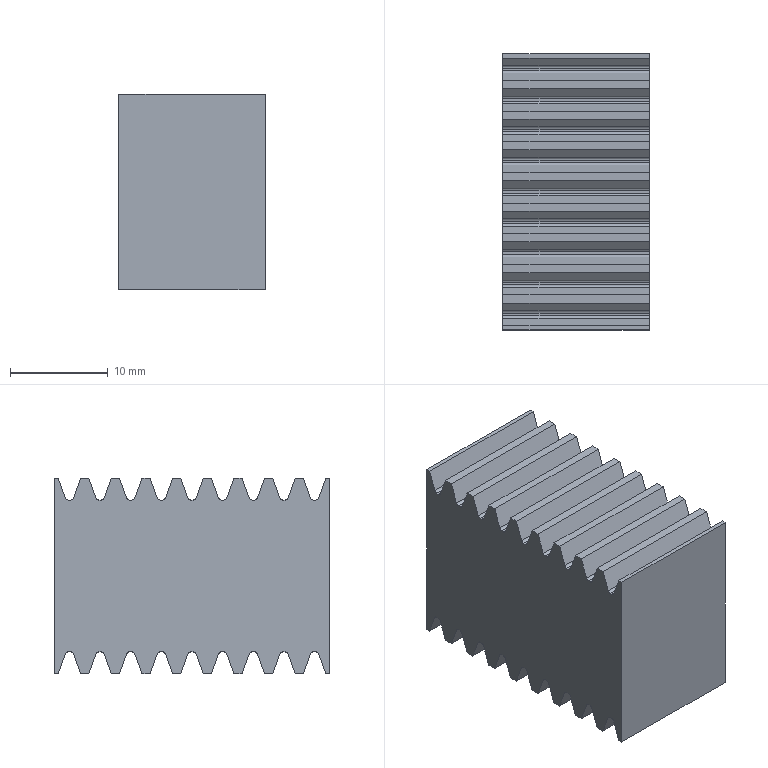Component | SolidWorks | ArmGrippingRack-1 | 1 solid | 117 faces | box 15.02 x 28.27 x 20.07 mm | volume 6038 mm3 | plane 79 | cylinder 38 | commonest cylinder face diameters 0.6 x36 10 x2
build123d program:
from build123d import *

# Parameters (mm, degrees)
EXTRUDECI_DEPTH                = 7.5
EXTRUDECI_DEPTH_BACK           = 7.5
SKETCHCI_M_STRSKETCHNAME_W     = 20.05
SKETCHCI_M_STRSKETCHNAME_H     = 69.115
TOOTHEXTRUDECUTSPURGEAR2_DEPTH = 7.5
PATTERNSPURGEAR2_COUNT         = 22
PATTERNSPURGEAR2_PITCH         = 3.142
MIRROR1_COPY_1_DEPTH           = 7.5
MIRROR1_COPY_2_DEPTH           = 7.5
MIRROR1_COPY_3_DEPTH           = 7.5
MIRROR1_COPY_4_DEPTH           = 7.5
MIRROR1_COPY_5_DEPTH           = 7.5
MIRROR1_COPY_6_DEPTH           = 7.5
MIRROR1_COPY_7_DEPTH           = 7.5
MIRROR1_COPY_8_DEPTH           = 7.5
MIRROR1_COPY_9_DEPTH           = 7.5
MIRROR1_COPY_10_DEPTH          = 7.5
MIRROR1_COPY_11_DEPTH          = 7.5
MIRROR1_COPY_12_DEPTH          = 7.5
MIRROR1_COPY_13_DEPTH          = 7.5
MIRROR1_COPY_14_DEPTH          = 7.5
MIRROR1_COPY_15_DEPTH          = 7.5
MIRROR1_COPY_16_DEPTH          = 7.5
MIRROR1_COPY_17_DEPTH          = 7.5
MIRROR1_COPY_18_DEPTH          = 7.5
MIRROR1_COPY_19_DEPTH          = 7.5
MIRROR1_COPY_20_DEPTH          = 7.5
MIRROR1_COPY_21_DEPTH          = 7.5
SKETCH4_W                      = 58.506
SKETCH4_H                      = 46.448
CUT_EXTRUDE2_DEPTH             = 20
SKETCH5_R                      = 5
CUT_EXTRUDE3_DEPTH             = 20


with BuildPart() as part:
    # SketchCI.m_strSketchName → ExtrudeCI (new, two sides: drawn at the far end of the back side and taken through both)
    with BuildSketch(Plane.XY.offset(-EXTRUDECI_DEPTH_BACK)):
        with Locations((9.025, -32.987)):
            Rectangle(SKETCHCI_M_STRSKETCHNAME_W, SKETCHCI_M_STRSKETCHNAME_H)
    extrude(amount=EXTRUDECI_DEPTH + EXTRUDECI_DEPTH_BACK)

    # SketchToothSpurGear2 → ToothExtrudeCutSpurGear2 (cut, symmetric)
    with BuildSketch(Plane.XY):
        with BuildLine():
            Line((-1, 1.149), (-1, -1.149))
            Line((-1, -1.149), (1.053, -0.4023))
            ThreePointArc((1.053, -0.4023), (1.196, -0.2924), (1.25, -0.1204))
            Line((1.25, -0.1204), (1.25, 0.1204))
            ThreePointArc((1.25, 0.1204), (1.196, 0.2924), (1.053, 0.4023))
            Line((1.053, 0.4023), (-1, 1.149))
        make_face()
    toothextrudecutspurgear2 = extrude(amount=TOOTHEXTRUDECUTSPURGEAR2_DEPTH, both=True, mode=Mode.SUBTRACT)

    # PatternSpurGear2: ToothExtrudeCutSpurGear2 ×22
    with Locations(*[(0, -i * PATTERNSPURGEAR2_PITCH, 0) for i in range(1, PATTERNSPURGEAR2_COUNT)]):
        add(toothextrudecutspurgear2, mode=Mode.SUBTRACT)

    # Mirror1: ToothExtrudeCutSpurGear2 across plane
    add(toothextrudecutspurgear2.mirror(Plane(origin=(9.025, 0, 0), x_dir=(0, 0, 1), z_dir=(1, 0, 0))), mode=Mode.SUBTRACT)

    # Mirror1 copy 1 sketch → Mirror1 copy 1 (cut, symmetric)
    with BuildSketch(Plane(origin=(18.05, -3.142, 0), x_dir=(-1, 0, 0), z_dir=(0, 0, 1))):
        with BuildLine():
            Line((-1, -1.149), (-1, 1.149))
            Line((-1, 1.149), (1.053, 0.4023))
            ThreePointArc((1.053, 0.4023), (1.196, 0.2924), (1.25, 0.1204))
            Line((1.25, 0.1204), (1.25, -0.1204))
            ThreePointArc((1.25, -0.1204), (1.196, -0.2924), (1.053, -0.4023))
            Line((1.053, -0.4023), (-1, -1.149))
        make_face()
    extrude(amount=MIRROR1_COPY_1_DEPTH, both=True, mode=Mode.SUBTRACT)

    # Mirror1 copy 2 sketch → Mirror1 copy 2 (cut, symmetric)
    with BuildSketch(Plane(origin=(18.05, -6.283, 0), x_dir=(-1, 0, 0), z_dir=(0, 0, 1))):
        with BuildLine():
            Line((-1, -1.149), (-1, 1.149))
            Line((-1, 1.149), (1.053, 0.4023))
            ThreePointArc((1.053, 0.4023), (1.196, 0.2924), (1.25, 0.1204))
            Line((1.25, 0.1204), (1.25, -0.1204))
            ThreePointArc((1.25, -0.1204), (1.196, -0.2924), (1.053, -0.4023))
            Line((1.053, -0.4023), (-1, -1.149))
        make_face()
    extrude(amount=MIRROR1_COPY_2_DEPTH, both=True, mode=Mode.SUBTRACT)

    # Mirror1 copy 3 sketch → Mirror1 copy 3 (cut, symmetric)
    with BuildSketch(Plane(origin=(18.05, -9.425, 0), x_dir=(-1, 0, 0), z_dir=(0, 0, 1))):
        with BuildLine():
            Line((-1, -1.149), (-1, 1.149))
            Line((-1, 1.149), (1.053, 0.4023))
            ThreePointArc((1.053, 0.4023), (1.196, 0.2924), (1.25, 0.1204))
            Line((1.25, 0.1204), (1.25, -0.1204))
            ThreePointArc((1.25, -0.1204), (1.196, -0.2924), (1.053, -0.4023))
            Line((1.053, -0.4023), (-1, -1.149))
        make_face()
    extrude(amount=MIRROR1_COPY_3_DEPTH, both=True, mode=Mode.SUBTRACT)

    # Mirror1 copy 4 sketch → Mirror1 copy 4 (cut, symmetric)
    with BuildSketch(Plane(origin=(18.05, -12.566, 0), x_dir=(-1, 0, 0), z_dir=(0, 0, 1))):
        with BuildLine():
            Line((-1, -1.149), (-1, 1.149))
            Line((-1, 1.149), (1.053, 0.4023))
            ThreePointArc((1.053, 0.4023), (1.196, 0.2924), (1.25, 0.1204))
            Line((1.25, 0.1204), (1.25, -0.1204))
            ThreePointArc((1.25, -0.1204), (1.196, -0.2924), (1.053, -0.4023))
            Line((1.053, -0.4023), (-1, -1.149))
        make_face()
    extrude(amount=MIRROR1_COPY_4_DEPTH, both=True, mode=Mode.SUBTRACT)

    # Mirror1 copy 5 sketch → Mirror1 copy 5 (cut, symmetric)
    with BuildSketch(Plane(origin=(18.05, -15.708, 0), x_dir=(-1, 0, 0), z_dir=(0, 0, 1))):
        with BuildLine():
            Line((-1, -1.149), (-1, 1.149))
            Line((-1, 1.149), (1.053, 0.4023))
            ThreePointArc((1.053, 0.4023), (1.196, 0.2924), (1.25, 0.1204))
            Line((1.25, 0.1204), (1.25, -0.1204))
            ThreePointArc((1.25, -0.1204), (1.196, -0.2924), (1.053, -0.4023))
            Line((1.053, -0.4023), (-1, -1.149))
        make_face()
    extrude(amount=MIRROR1_COPY_5_DEPTH, both=True, mode=Mode.SUBTRACT)

    # Mirror1 copy 6 sketch → Mirror1 copy 6 (cut, symmetric)
    with BuildSketch(Plane(origin=(18.05, -18.85, 0), x_dir=(-1, 0, 0), z_dir=(0, 0, 1))):
        with BuildLine():
            Line((-1, -1.149), (-1, 1.149))
            Line((-1, 1.149), (1.053, 0.4023))
            ThreePointArc((1.053, 0.4023), (1.196, 0.2924), (1.25, 0.1204))
            Line((1.25, 0.1204), (1.25, -0.1204))
            ThreePointArc((1.25, -0.1204), (1.196, -0.2924), (1.053, -0.4023))
            Line((1.053, -0.4023), (-1, -1.149))
        make_face()
    extrude(amount=MIRROR1_COPY_6_DEPTH, both=True, mode=Mode.SUBTRACT)

    # Mirror1 copy 7 sketch → Mirror1 copy 7 (cut, symmetric)
    with BuildSketch(Plane(origin=(18.05, -21.991, 0), x_dir=(-1, 0, 0), z_dir=(0, 0, 1))):
        with BuildLine():
            Line((-1, -1.149), (-1, 1.149))
            Line((-1, 1.149), (1.053, 0.4023))
            ThreePointArc((1.053, 0.4023), (1.196, 0.2924), (1.25, 0.1204))
            Line((1.25, 0.1204), (1.25, -0.1204))
            ThreePointArc((1.25, -0.1204), (1.196, -0.2924), (1.053, -0.4023))
            Line((1.053, -0.4023), (-1, -1.149))
        make_face()
    extrude(amount=MIRROR1_COPY_7_DEPTH, both=True, mode=Mode.SUBTRACT)

    # Mirror1 copy 8 sketch → Mirror1 copy 8 (cut, symmetric)
    with BuildSketch(Plane(origin=(18.05, -25.133, 0), x_dir=(-1, 0, 0), z_dir=(0, 0, 1))):
        with BuildLine():
            Line((-1, -1.149), (-1, 1.149))
            Line((-1, 1.149), (1.053, 0.4023))
            ThreePointArc((1.053, 0.4023), (1.196, 0.2924), (1.25, 0.1204))
            Line((1.25, 0.1204), (1.25, -0.1204))
            ThreePointArc((1.25, -0.1204), (1.196, -0.2924), (1.053, -0.4023))
            Line((1.053, -0.4023), (-1, -1.149))
        make_face()
    extrude(amount=MIRROR1_COPY_8_DEPTH, both=True, mode=Mode.SUBTRACT)

    # Mirror1 copy 9 sketch → Mirror1 copy 9 (cut, symmetric)
    with BuildSketch(Plane(origin=(18.05, -28.274, 0), x_dir=(-1, 0, 0), z_dir=(0, 0, 1))):
        with BuildLine():
            Line((-1, -1.149), (-1, 1.149))
            Line((-1, 1.149), (1.053, 0.4023))
            ThreePointArc((1.053, 0.4023), (1.196, 0.2924), (1.25, 0.1204))
            Line((1.25, 0.1204), (1.25, -0.1204))
            ThreePointArc((1.25, -0.1204), (1.196, -0.2924), (1.053, -0.4023))
            Line((1.053, -0.4023), (-1, -1.149))
        make_face()
    extrude(amount=MIRROR1_COPY_9_DEPTH, both=True, mode=Mode.SUBTRACT)

    # Mirror1 copy 10 sketch → Mirror1 copy 10 (cut, symmetric)
    with BuildSketch(Plane(origin=(18.05, -31.416, 0), x_dir=(-1, 0, 0), z_dir=(0, 0, 1))):
        with BuildLine():
            Line((-1, -1.149), (-1, 1.149))
            Line((-1, 1.149), (1.053, 0.4023))
            ThreePointArc((1.053, 0.4023), (1.196, 0.2924), (1.25, 0.1204))
            Line((1.25, 0.1204), (1.25, -0.1204))
            ThreePointArc((1.25, -0.1204), (1.196, -0.2924), (1.053, -0.4023))
            Line((1.053, -0.4023), (-1, -1.149))
        make_face()
    extrude(amount=MIRROR1_COPY_10_DEPTH, both=True, mode=Mode.SUBTRACT)

    # Mirror1 copy 11 sketch → Mirror1 copy 11 (cut, symmetric)
    with BuildSketch(Plane(origin=(18.05, -34.558, 0), x_dir=(-1, 0, 0), z_dir=(0, 0, 1))):
        with BuildLine():
            Line((-1, -1.149), (-1, 1.149))
            Line((-1, 1.149), (1.053, 0.4023))
            ThreePointArc((1.053, 0.4023), (1.196, 0.2924), (1.25, 0.1204))
            Line((1.25, 0.1204), (1.25, -0.1204))
            ThreePointArc((1.25, -0.1204), (1.196, -0.2924), (1.053, -0.4023))
            Line((1.053, -0.4023), (-1, -1.149))
        make_face()
    extrude(amount=MIRROR1_COPY_11_DEPTH, both=True, mode=Mode.SUBTRACT)

    # Mirror1 copy 12 sketch → Mirror1 copy 12 (cut, symmetric)
    with BuildSketch(Plane(origin=(18.05, -37.699, 0), x_dir=(-1, 0, 0), z_dir=(0, 0, 1))):
        with BuildLine():
            Line((-1, -1.149), (-1, 1.149))
            Line((-1, 1.149), (1.053, 0.4023))
            ThreePointArc((1.053, 0.4023), (1.196, 0.2924), (1.25, 0.1204))
            Line((1.25, 0.1204), (1.25, -0.1204))
            ThreePointArc((1.25, -0.1204), (1.196, -0.2924), (1.053, -0.4023))
            Line((1.053, -0.4023), (-1, -1.149))
        make_face()
    extrude(amount=MIRROR1_COPY_12_DEPTH, both=True, mode=Mode.SUBTRACT)

    # Mirror1 copy 13 sketch → Mirror1 copy 13 (cut, symmetric)
    with BuildSketch(Plane(origin=(18.05, -40.841, 0), x_dir=(-1, 0, 0), z_dir=(0, 0, 1))):
        with BuildLine():
            Line((-1, -1.149), (-1, 1.149))
            Line((-1, 1.149), (1.053, 0.4023))
            ThreePointArc((1.053, 0.4023), (1.196, 0.2924), (1.25, 0.1204))
            Line((1.25, 0.1204), (1.25, -0.1204))
            ThreePointArc((1.25, -0.1204), (1.196, -0.2924), (1.053, -0.4023))
            Line((1.053, -0.4023), (-1, -1.149))
        make_face()
    extrude(amount=MIRROR1_COPY_13_DEPTH, both=True, mode=Mode.SUBTRACT)

    # Mirror1 copy 14 sketch → Mirror1 copy 14 (cut, symmetric)
    with BuildSketch(Plane(origin=(18.05, -43.982, 0), x_dir=(-1, 0, 0), z_dir=(0, 0, 1))):
        with BuildLine():
            Line((-1, -1.149), (-1, 1.149))
            Line((-1, 1.149), (1.053, 0.4023))
            ThreePointArc((1.053, 0.4023), (1.196, 0.2924), (1.25, 0.1204))
            Line((1.25, 0.1204), (1.25, -0.1204))
            ThreePointArc((1.25, -0.1204), (1.196, -0.2924), (1.053, -0.4023))
            Line((1.053, -0.4023), (-1, -1.149))
        make_face()
    extrude(amount=MIRROR1_COPY_14_DEPTH, both=True, mode=Mode.SUBTRACT)

    # Mirror1 copy 15 sketch → Mirror1 copy 15 (cut, symmetric)
    with BuildSketch(Plane(origin=(18.05, -47.124, 0), x_dir=(-1, 0, 0), z_dir=(0, 0, 1))):
        with BuildLine():
            Line((-1, -1.149), (-1, 1.149))
            Line((-1, 1.149), (1.053, 0.4023))
            ThreePointArc((1.053, 0.4023), (1.196, 0.2924), (1.25, 0.1204))
            Line((1.25, 0.1204), (1.25, -0.1204))
            ThreePointArc((1.25, -0.1204), (1.196, -0.2924), (1.053, -0.4023))
            Line((1.053, -0.4023), (-1, -1.149))
        make_face()
    extrude(amount=MIRROR1_COPY_15_DEPTH, both=True, mode=Mode.SUBTRACT)

    # Mirror1 copy 16 sketch → Mirror1 copy 16 (cut, symmetric)
    with BuildSketch(Plane(origin=(18.05, -50.265, 0), x_dir=(-1, 0, 0), z_dir=(0, 0, 1))):
        with BuildLine():
            Line((-1, -1.149), (-1, 1.149))
            Line((-1, 1.149), (1.053, 0.4023))
            ThreePointArc((1.053, 0.4023), (1.196, 0.2924), (1.25, 0.1204))
            Line((1.25, 0.1204), (1.25, -0.1204))
            ThreePointArc((1.25, -0.1204), (1.196, -0.2924), (1.053, -0.4023))
            Line((1.053, -0.4023), (-1, -1.149))
        make_face()
    extrude(amount=MIRROR1_COPY_16_DEPTH, both=True, mode=Mode.SUBTRACT)

    # Mirror1 copy 17 sketch → Mirror1 copy 17 (cut, symmetric)
    with BuildSketch(Plane(origin=(18.05, -53.407, 0), x_dir=(-1, 0, 0), z_dir=(0, 0, 1))):
        with BuildLine():
            Line((-1, -1.149), (-1, 1.149))
            Line((-1, 1.149), (1.053, 0.4023))
            ThreePointArc((1.053, 0.4023), (1.196, 0.2924), (1.25, 0.1204))
            Line((1.25, 0.1204), (1.25, -0.1204))
            ThreePointArc((1.25, -0.1204), (1.196, -0.2924), (1.053, -0.4023))
            Line((1.053, -0.4023), (-1, -1.149))
        make_face()
    extrude(amount=MIRROR1_COPY_17_DEPTH, both=True, mode=Mode.SUBTRACT)

    # Mirror1 copy 18 sketch → Mirror1 copy 18 (cut, symmetric)
    with BuildSketch(Plane(origin=(18.05, -56.549, 0), x_dir=(-1, 0, 0), z_dir=(0, 0, 1))):
        with BuildLine():
            Line((-1, -1.149), (-1, 1.149))
            Line((-1, 1.149), (1.053, 0.4023))
            ThreePointArc((1.053, 0.4023), (1.196, 0.2924), (1.25, 0.1204))
            Line((1.25, 0.1204), (1.25, -0.1204))
            ThreePointArc((1.25, -0.1204), (1.196, -0.2924), (1.053, -0.4023))
            Line((1.053, -0.4023), (-1, -1.149))
        make_face()
    extrude(amount=MIRROR1_COPY_18_DEPTH, both=True, mode=Mode.SUBTRACT)

    # Mirror1 copy 19 sketch → Mirror1 copy 19 (cut, symmetric)
    with BuildSketch(Plane(origin=(18.05, -59.69, 0), x_dir=(-1, 0, 0), z_dir=(0, 0, 1))):
        with BuildLine():
            Line((-1, -1.149), (-1, 1.149))
            Line((-1, 1.149), (1.053, 0.4023))
            ThreePointArc((1.053, 0.4023), (1.196, 0.2924), (1.25, 0.1204))
            Line((1.25, 0.1204), (1.25, -0.1204))
            ThreePointArc((1.25, -0.1204), (1.196, -0.2924), (1.053, -0.4023))
            Line((1.053, -0.4023), (-1, -1.149))
        make_face()
    extrude(amount=MIRROR1_COPY_19_DEPTH, both=True, mode=Mode.SUBTRACT)

    # Mirror1 copy 20 sketch → Mirror1 copy 20 (cut, symmetric)
    with BuildSketch(Plane(origin=(18.05, -62.832, 0), x_dir=(-1, 0, 0), z_dir=(0, 0, 1))):
        with BuildLine():
            Line((-1, -1.149), (-1, 1.149))
            Line((-1, 1.149), (1.053, 0.4023))
            ThreePointArc((1.053, 0.4023), (1.196, 0.2924), (1.25, 0.1204))
            Line((1.25, 0.1204), (1.25, -0.1204))
            ThreePointArc((1.25, -0.1204), (1.196, -0.2924), (1.053, -0.4023))
            Line((1.053, -0.4023), (-1, -1.149))
        make_face()
    extrude(amount=MIRROR1_COPY_20_DEPTH, both=True, mode=Mode.SUBTRACT)

    # Mirror1 copy 21 sketch → Mirror1 copy 21 (cut, symmetric)
    with BuildSketch(Plane(origin=(18.05, -65.973, 0), x_dir=(-1, 0, 0), z_dir=(0, 0, 1))):
        with BuildLine():
            Line((-1, -1.149), (-1, 1.149))
            Line((-1, 1.149), (1.053, 0.4023))
            ThreePointArc((1.053, 0.4023), (1.196, 0.2924), (1.25, 0.1204))
            Line((1.25, 0.1204), (1.25, -0.1204))
            ThreePointArc((1.25, -0.1204), (1.196, -0.2924), (1.053, -0.4023))
            Line((1.053, -0.4023), (-1, -1.149))
        make_face()
    extrude(amount=MIRROR1_COPY_21_DEPTH, both=True, mode=Mode.SUBTRACT)

    # Sketch4 → Cut-Extrude2 (cut)
    with BuildSketch(Plane.XY.offset(7.5)):
        with Locations((12.115, -49.928)):
            Rectangle(SKETCH4_W, SKETCH4_H)
    extrude(amount=-CUT_EXTRUDE2_DEPTH, mode=Mode.SUBTRACT)

    # Sketch5 → Cut-Extrude3 (cut)
    with BuildSketch(Plane(origin=(0, 1.571, 0), x_dir=(1, 0, 0), z_dir=(0, 1, 0))):
        with Locations(Location((9.025, 0, 0), (0, 0, 270))):
            Circle(SKETCH5_R)
    extrude(amount=-CUT_EXTRUDE3_DEPTH, mode=Mode.SUBTRACT)


solid = part.part

# Placed as in the assembly
solid = solid.moved(Location((-125.052, 775.395, 1100.728), (0, -89.938, 0)))